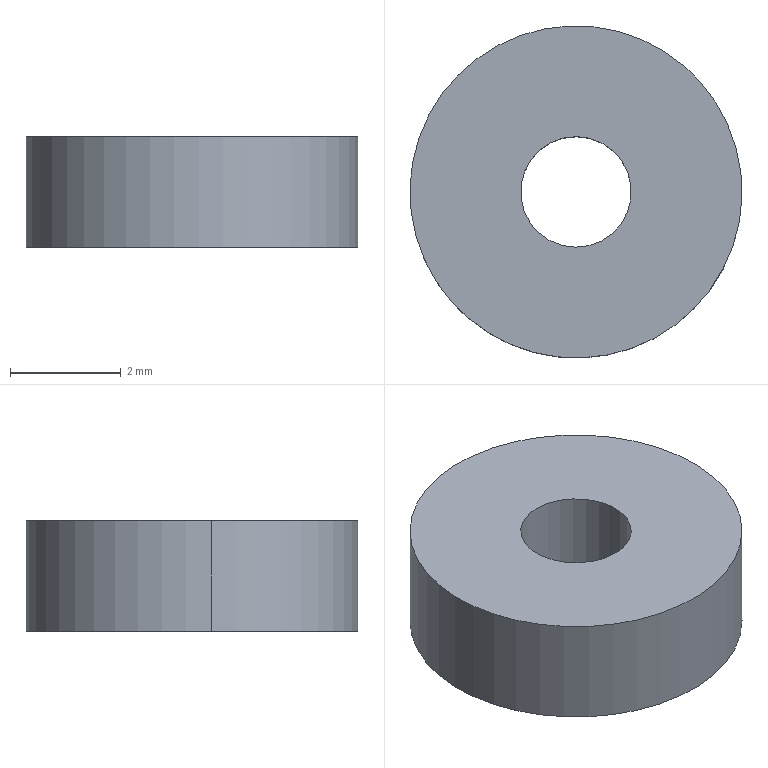Component | SolidWorks | RearAxisWasher-2 | 1 solid | 6 faces | box 6 x 6 x 2 mm | volume 50 mm3 | cylinder 4 | plane 2 | commonest cylinder face diameters 2 x2 6 x2
build123d program:
from build123d import *

# Parameters (mm, degrees)
SKETCH1_R           = 3
SKETCH1_R_2         = 1
BOSS_EXTRUDE1_DEPTH = 2


with BuildPart() as part:
    # Sketch1 → Boss-Extrude1 (new body)
    with BuildSketch(Plane.XY):
        with Locations((-16, -3.5)):
            Circle(SKETCH1_R)
        with Locations((-16, -3.5)):
            Circle(SKETCH1_R_2, mode=Mode.SUBTRACT)
    extrude(amount=BOSS_EXTRUDE1_DEPTH)


solid = part.part

# Placed as in the assembly
solid = solid.moved(Location((28.5, 0, -3), (0, 0, 0)))
STEP:
#1=CARTESIAN_POINT('',(0.453,-0.1423,-0.03937));
#2=VERTEX_POINT('',#1);
#3=CARTESIAN_POINT('',(0.5312,-0.1332,-0.03937));
#4=VERTEX_POINT('',#3);
#5=CARTESIAN_POINT('',(0.4921,-0.1378,-0.03937));
#6=DIRECTION('',(-0.,-0.,1.));
#7=DIRECTION('',(0.9933,0.1155,0.));
#8=AXIS2_PLACEMENT_3D('',#5,#6,#7);
#9=CIRCLE('',#8,0.03937);
#10=EDGE_CURVE('',#2,#4,#9,.T.);
#11=ORIENTED_EDGE('',*,*,#10,.T.);
#12=CARTESIAN_POINT('',(0.5312,-0.1332,-0.1181));
#13=VERTEX_POINT('',#12);
#14=CARTESIAN_POINT('',(0.5312,-0.1332,-0.03937));
#15=DIRECTION('',(0.,0.,-1.));
#16=VECTOR('',#15,39.37);
#17=LINE('',#14,#16);
#18=EDGE_CURVE('',#4,#13,#17,.T.);
#19=ORIENTED_EDGE('',*,*,#18,.T.);
#20=CARTESIAN_POINT('',(0.453,-0.1423,-0.1181));
#21=VERTEX_POINT('',#20);
#22=CARTESIAN_POINT('',(0.4921,-0.1378,-0.1181));
#23=DIRECTION('',(-0.,-0.,1.));
#24=DIRECTION('',(0.9933,0.1155,0.));
#25=AXIS2_PLACEMENT_3D('',#22,#23,#24);
#26=CIRCLE('',#25,0.03937);
#27=EDGE_CURVE('',#21,#13,#26,.T.);
#28=ORIENTED_EDGE('',*,*,#27,.F.);
#29=CARTESIAN_POINT('',(0.453,-0.1423,-0.03937));
#30=DIRECTION('',(0.,0.,-1.));
#31=VECTOR('',#30,39.37);
#32=LINE('',#29,#31);
#33=EDGE_CURVE('',#2,#21,#32,.T.);
#34=ORIENTED_EDGE('',*,*,#33,.F.);
#35=EDGE_LOOP('',(#11,#19,#28,#34));
#36=FACE_OUTER_BOUND('',#35,.T.);
#37=CARTESIAN_POINT('',(0.4921,-0.1378,-0.03937));
#38=DIRECTION('',(0.,0.,-1.));
#39=DIRECTION('',(-0.9933,-0.1155,-0.));
#40=AXIS2_PLACEMENT_3D('',#37,#38,#39);
#41=CYLINDRICAL_SURFACE('',#40,0.03937);
#42=ADVANCED_FACE('',(#36),#41,.F.);
#43=CARTESIAN_POINT('',(0.6094,-0.1242,-0.03937));
#44=VERTEX_POINT('',#43);
#45=CARTESIAN_POINT('',(0.3748,-0.1514,-0.03937));
#46=VERTEX_POINT('',#45);
#47=CARTESIAN_POINT('',(0.4921,-0.1378,-0.03937));
#48=DIRECTION('',(-0.,-0.,1.));
#49=DIRECTION('',(0.9933,0.1155,0.));
#50=AXIS2_PLACEMENT_3D('',#47,#48,#49);
#51=CIRCLE('',#50,0.1181);
#52=EDGE_CURVE('',#44,#46,#51,.T.);
#53=ORIENTED_EDGE('',*,*,#52,.F.);
#54=CARTESIAN_POINT('',(0.6094,-0.1242,-0.1181));
#55=VERTEX_POINT('',#54);
#56=CARTESIAN_POINT('',(0.6094,-0.1242,-0.03937));
#57=DIRECTION('',(0.,0.,-1.));
#58=VECTOR('',#57,39.37);
#59=LINE('',#56,#58);
#60=EDGE_CURVE('',#44,#55,#59,.T.);
#61=ORIENTED_EDGE('',*,*,#60,.T.);
#62=CARTESIAN_POINT('',(0.3748,-0.1514,-0.1181));
#63=VERTEX_POINT('',#62);
#64=CARTESIAN_POINT('',(0.4921,-0.1378,-0.1181));
#65=DIRECTION('',(-0.,-0.,1.));
#66=DIRECTION('',(0.9933,0.1155,0.));
#67=AXIS2_PLACEMENT_3D('',#64,#65,#66);
#68=CIRCLE('',#67,0.1181);
#69=EDGE_CURVE('',#55,#63,#68,.T.);
#70=ORIENTED_EDGE('',*,*,#69,.T.);
#71=CARTESIAN_POINT('',(0.3748,-0.1514,-0.03937));
#72=DIRECTION('',(0.,0.,-1.));
#73=VECTOR('',#72,39.37);
#74=LINE('',#71,#73);
#75=EDGE_CURVE('',#46,#63,#74,.T.);
#76=ORIENTED_EDGE('',*,*,#75,.F.);
#77=EDGE_LOOP('',(#53,#61,#70,#76));
#78=FACE_OUTER_BOUND('',#77,.T.);
#79=CARTESIAN_POINT('',(0.4921,-0.1378,-0.03937));
#80=DIRECTION('',(0.,0.,-1.));
#81=DIRECTION('',(-0.9933,-0.1155,-0.));
#82=AXIS2_PLACEMENT_3D('',#79,#80,#81);
#83=CYLINDRICAL_SURFACE('',#82,0.1181);
#84=ADVANCED_FACE('',(#78),#83,.T.);
#85=CARTESIAN_POINT('',(0.4921,-0.1378,-0.03937));
#86=DIRECTION('',(-0.,-0.,1.));
#87=DIRECTION('',(0.9933,0.1155,0.));
#88=AXIS2_PLACEMENT_3D('',#85,#86,#87);
#89=CIRCLE('',#88,0.1181);
#90=EDGE_CURVE('',#46,#44,#89,.T.);
#91=ORIENTED_EDGE('',*,*,#90,.T.);
#92=ORIENTED_EDGE('',*,*,#52,.T.);
#93=EDGE_LOOP('',(#91,#92));
#94=FACE_OUTER_BOUND('',#93,.T.);
#95=ORIENTED_EDGE('',*,*,#10,.F.);
#96=CARTESIAN_POINT('',(0.4921,-0.1378,-0.03937));
#97=DIRECTION('',(-0.,-0.,1.));
#98=DIRECTION('',(0.9933,0.1155,0.));
#99=AXIS2_PLACEMENT_3D('',#96,#97,#98);
#100=CIRCLE('',#99,0.03937);
#101=EDGE_CURVE('',#4,#2,#100,.T.);
#102=ORIENTED_EDGE('',*,*,#101,.F.);
#103=EDGE_LOOP('',(#95,#102));
#104=FACE_BOUND('',#103,.T.);
#105=CARTESIAN_POINT('',(0.4921,-0.1378,-0.03937));
#106=DIRECTION('',(-0.,-0.,1.));
#107=DIRECTION('',(0.9933,0.1155,0.));
#108=AXIS2_PLACEMENT_3D('',#105,#106,#107);
#109=PLANE('',#108);
#110=ADVANCED_FACE('',(#94,#104),#109,.T.);
#111=CARTESIAN_POINT('',(0.4921,-0.1378,-0.1181));
#112=DIRECTION('',(-0.,-0.,1.));
#113=DIRECTION('',(0.9933,0.1155,0.));
#114=AXIS2_PLACEMENT_3D('',#111,#112,#113);
#115=CIRCLE('',#114,0.1181);
#116=EDGE_CURVE('',#63,#55,#115,.T.);
#117=ORIENTED_EDGE('',*,*,#116,.F.);
#118=ORIENTED_EDGE('',*,*,#69,.F.);
#119=EDGE_LOOP('',(#117,#118));
#120=FACE_OUTER_BOUND('',#119,.T.);
#121=ORIENTED_EDGE('',*,*,#27,.T.);
#122=CARTESIAN_POINT('',(0.4921,-0.1378,-0.1181));
#123=DIRECTION('',(-0.,-0.,1.));
#124=DIRECTION('',(0.9933,0.1155,0.));
#125=AXIS2_PLACEMENT_3D('',#122,#123,#124);
#126=CIRCLE('',#125,0.03937);
#127=EDGE_CURVE('',#13,#21,#126,.T.);
#128=ORIENTED_EDGE('',*,*,#127,.T.);
#129=EDGE_LOOP('',(#121,#128));
#130=FACE_BOUND('',#129,.T.);
#131=CARTESIAN_POINT('',(0.4921,-0.1378,-0.1181));
#132=DIRECTION('',(-0.,-0.,1.));
#133=DIRECTION('',(0.9933,0.1155,0.));
#134=AXIS2_PLACEMENT_3D('',#131,#132,#133);
#135=PLANE('',#134);
#136=ADVANCED_FACE('',(#120,#130),#135,.F.);
#137=ORIENTED_EDGE('',*,*,#60,.F.);
#138=ORIENTED_EDGE('',*,*,#90,.F.);
#139=ORIENTED_EDGE('',*,*,#75,.T.);
#140=ORIENTED_EDGE('',*,*,#116,.T.);
#141=EDGE_LOOP('',(#137,#138,#139,#140));
#142=FACE_OUTER_BOUND('',#141,.T.);
#143=CARTESIAN_POINT('',(0.4921,-0.1378,-0.03937));
#144=DIRECTION('',(0.,0.,-1.));
#145=DIRECTION('',(-0.9933,-0.1155,-0.));
#146=AXIS2_PLACEMENT_3D('',#143,#144,#145);
#147=CYLINDRICAL_SURFACE('',#146,0.1181);
#148=ADVANCED_FACE('',(#142),#147,.T.);
#149=ORIENTED_EDGE('',*,*,#18,.F.);
#150=ORIENTED_EDGE('',*,*,#101,.T.);
#151=ORIENTED_EDGE('',*,*,#33,.T.);
#152=ORIENTED_EDGE('',*,*,#127,.F.);
#153=EDGE_LOOP('',(#149,#150,#151,#152));
#154=FACE_OUTER_BOUND('',#153,.T.);
#155=CARTESIAN_POINT('',(0.4921,-0.1378,-0.03937));
#156=DIRECTION('',(0.,0.,-1.));
#157=DIRECTION('',(-0.9933,-0.1155,-0.));
#158=AXIS2_PLACEMENT_3D('',#155,#156,#157);
#159=CYLINDRICAL_SURFACE('',#158,0.03937);
#160=ADVANCED_FACE('',(#154),#159,.F.);
#161=CLOSED_SHELL('',(#42,#84,#110,#136,#148,#160));
#162=MANIFOLD_SOLID_BREP('',#161);
#163=CARTESIAN_POINT('',(0.,0.,0.));
#164=DIRECTION('',(0.,0.,1.));
#165=DIRECTION('',(1.,0.,0.));
#166=AXIS2_PLACEMENT_3D('',#163,#164,#165);
#167=(LENGTH_UNIT()NAMED_UNIT(*)SI_UNIT($,.METRE.));
#168=LENGTH_MEASURE_WITH_UNIT(LENGTH_MEASURE(0.0254),#167);
#169=DIMENSIONAL_EXPONENTS(1.,0.,0.,0.,0.,0.,0.);
#170=(CONVERSION_BASED_UNIT('',#168)LENGTH_UNIT()NAMED_UNIT(#169));
#171=UNCERTAINTY_MEASURE_WITH_UNIT(LENGTH_MEASURE(0.00001),#170,'','');
#172=(NAMED_UNIT(*)PLANE_ANGLE_UNIT()SI_UNIT($,.RADIAN.));
#173=(NAMED_UNIT(*)SI_UNIT($,.STERADIAN.)SOLID_ANGLE_UNIT());
#174=(GEOMETRIC_REPRESENTATION_CONTEXT(3)GLOBAL_UNCERTAINTY_ASSIGNED_CONTEXT((#171))GLOBAL_UNIT_ASSIGNED_CONTEXT((#170,#172,#173))REPRESENTATION_CONTEXT('',''));
#175=ADVANCED_BREP_SHAPE_REPRESENTATION('',(#162,#166),#174);
#176=COLOUR_RGB('',0.7922,0.8196,0.9333);
#177=FILL_AREA_STYLE_COLOUR('',#176);
#178=FILL_AREA_STYLE('',(#177));
#179=SURFACE_STYLE_FILL_AREA(#178);
#180=SURFACE_SIDE_STYLE('',(#179));
#181=SURFACE_STYLE_USAGE(.BOTH.,#180);
#182=PRESENTATION_STYLE_ASSIGNMENT((#181));
#183=STYLED_ITEM('',(#182),#162);
#184=(LENGTH_UNIT()NAMED_UNIT(*)SI_UNIT($,.METRE.));
#185=LENGTH_MEASURE_WITH_UNIT(LENGTH_MEASURE(0.0254),#184);
#186=DIMENSIONAL_EXPONENTS(1.,0.,0.,0.,0.,0.,0.);
#187=(CONVERSION_BASED_UNIT('',#185)LENGTH_UNIT()NAMED_UNIT(#186));
#188=UNCERTAINTY_MEASURE_WITH_UNIT(LENGTH_MEASURE(0.00001),#187,'','');
#189=(NAMED_UNIT(*)PLANE_ANGLE_UNIT()SI_UNIT($,.RADIAN.));
#190=(NAMED_UNIT(*)SI_UNIT($,.STERADIAN.)SOLID_ANGLE_UNIT());
#191=(GEOMETRIC_REPRESENTATION_CONTEXT(3)GLOBAL_UNCERTAINTY_ASSIGNED_CONTEXT((#188))GLOBAL_UNIT_ASSIGNED_CONTEXT((#187,#189,#190))REPRESENTATION_CONTEXT('',''));
#192=MECHANICAL_DESIGN_GEOMETRIC_PRESENTATION_REPRESENTATION('',(#183),#191);
#193=PRESENTATION_LAYER_ASSIGNMENT('','',(#183));